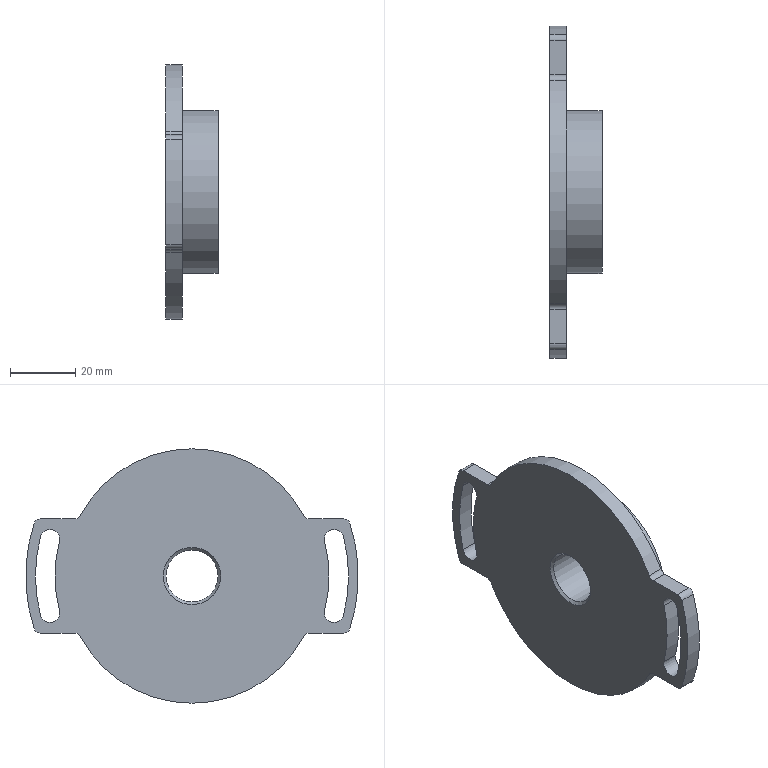Component | NX | END_CAP_2 | 1 solid | 31 faces | volume 44904 mm3 | cylinder 22 | plane 7 | cone 2 | commonest cylinder face diameters 4 x8 6 x4 102 x2 78 x2 96 x2 84 x2 50 x1 16 x1